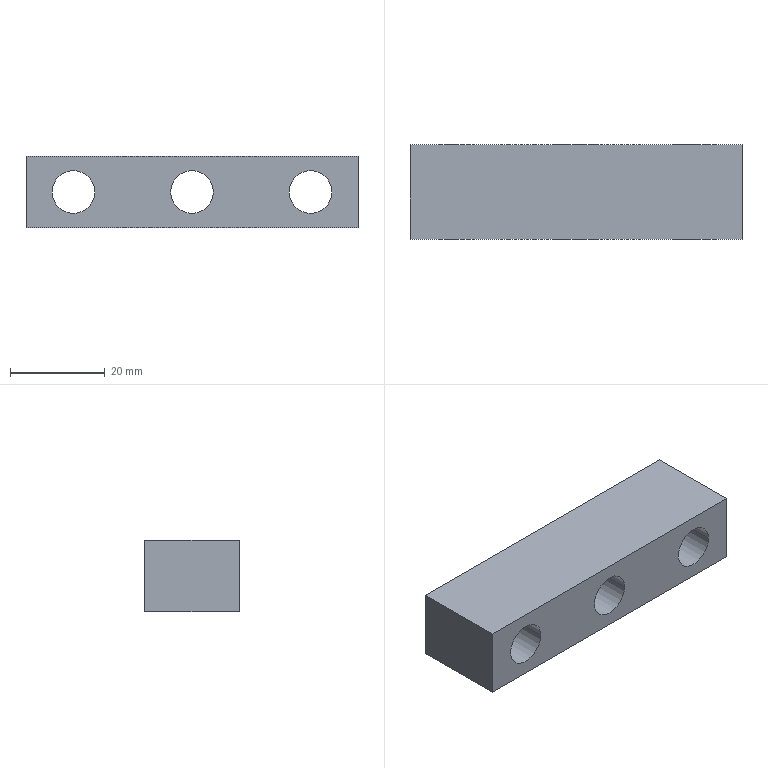Component | SolidWorks | -SpacerPlate-1 | 1 solid | 12 faces | box 70 x 20 x 15 mm | volume 17183 mm3 | cylinder 6 | plane 6 | commonest cylinder face diameters 9 x6
build123d program:
from build123d import *

# Parameters (mm, degrees)
SKETCH1_W                = 15
SKETCH1_H                = 70
BOSS_EXTRUDE1_DEPTH      = 20
F_9_0_9_DIAMETER_HOLE1_D = 9


with BuildPart() as part:
    # Sketch1 → Boss-Extrude1 (new body)
    with BuildSketch(Plane(origin=(0, 0, 0), x_dir=(1, 0, 0), z_dir=(0, 1, 0))):
        with Locations((-7.5, -35)):
            Rectangle(SKETCH1_W, SKETCH1_H)
    extrude(amount=BOSS_EXTRUDE1_DEPTH)

    # 9.0 _9_ Diameter Hole1 (through all)
    with Locations(Plane(origin=(0, 20, 0), x_dir=(1, 0, 0), z_dir=(0, 1, 0))):
        with Locations((-7.5, -10), (-7.5, -35), (-7.5, -60)):
            Hole(F_9_0_9_DIAMETER_HOLE1_D / 2)


solid = part.part

# Placed as in the assembly
solid = solid.moved(Location((170, 1289.5, -85), (0, 90, 0)))
STEP:
#1=COLOUR_RGB('',0.7922,0.8196,0.9333);
#2=FILL_AREA_STYLE_COLOUR('',#1);
#3=FILL_AREA_STYLE('',(#2));
#4=SURFACE_STYLE_FILL_AREA(#3);
#5=SURFACE_SIDE_STYLE('',(#4));
#6=SURFACE_STYLE_USAGE(.BOTH.,#5);
#7=PRESENTATION_STYLE_ASSIGNMENT((#6));
#8=CARTESIAN_POINT('',(9.232,50.768,-3.051));
#9=VERTEX_POINT('',#8);
#10=CARTESIAN_POINT('',(8.878,50.768,-3.051));
#11=VERTEX_POINT('',#10);
#12=CARTESIAN_POINT('',(9.055,50.768,-3.051));
#13=DIRECTION('',(0.,1.,0.));
#14=DIRECTION('',(-1.,0.,0.));
#15=AXIS2_PLACEMENT_3D('',#12,#13,#14);
#16=CIRCLE('',#15,0.1772);
#17=EDGE_CURVE('',#9,#11,#16,.T.);
#18=ORIENTED_EDGE('',*,*,#17,.F.);
#19=CARTESIAN_POINT('',(9.232,51.555,-3.051));
#20=VERTEX_POINT('',#19);
#21=CARTESIAN_POINT('',(9.232,51.555,-3.051));
#22=DIRECTION('',(0.,1.,0.));
#23=VECTOR('',#22,39.37);
#24=LINE('',#21,#23);
#25=EDGE_CURVE('',#9,#20,#24,.T.);
#26=ORIENTED_EDGE('',*,*,#25,.T.);
#27=CARTESIAN_POINT('',(8.878,51.555,-3.051));
#28=VERTEX_POINT('',#27);
#29=CARTESIAN_POINT('',(9.055,51.555,-3.051));
#30=DIRECTION('',(0.,1.,0.));
#31=DIRECTION('',(-1.,0.,0.));
#32=AXIS2_PLACEMENT_3D('',#29,#30,#31);
#33=CIRCLE('',#32,0.1772);
#34=EDGE_CURVE('',#20,#28,#33,.T.);
#35=ORIENTED_EDGE('',*,*,#34,.T.);
#36=CARTESIAN_POINT('',(8.878,51.555,-3.051));
#37=DIRECTION('',(0.,1.,0.));
#38=VECTOR('',#37,39.37);
#39=LINE('',#36,#38);
#40=EDGE_CURVE('',#11,#28,#39,.T.);
#41=ORIENTED_EDGE('',*,*,#40,.F.);
#42=EDGE_LOOP('',(#18,#26,#35,#41));
#43=FACE_OUTER_BOUND('',#42,.T.);
#44=CARTESIAN_POINT('',(9.055,51.555,-3.051));
#45=DIRECTION('',(0.,1.,0.));
#46=DIRECTION('',(-1.,0.,0.));
#47=AXIS2_PLACEMENT_3D('',#44,#45,#46);
#48=CYLINDRICAL_SURFACE('',#47,0.1772);
#49=ADVANCED_FACE('',(#43),#48,.F.);
#50=CARTESIAN_POINT('',(8.248,50.768,-3.051));
#51=VERTEX_POINT('',#50);
#52=CARTESIAN_POINT('',(7.894,50.768,-3.051));
#53=VERTEX_POINT('',#52);
#54=CARTESIAN_POINT('',(8.071,50.768,-3.051));
#55=DIRECTION('',(0.,1.,0.));
#56=DIRECTION('',(-1.,0.,0.));
#57=AXIS2_PLACEMENT_3D('',#54,#55,#56);
#58=CIRCLE('',#57,0.1772);
#59=EDGE_CURVE('',#51,#53,#58,.T.);
#60=ORIENTED_EDGE('',*,*,#59,.F.);
#61=CARTESIAN_POINT('',(8.248,51.555,-3.051));
#62=VERTEX_POINT('',#61);
#63=CARTESIAN_POINT('',(8.248,51.555,-3.051));
#64=DIRECTION('',(0.,1.,0.));
#65=VECTOR('',#64,39.37);
#66=LINE('',#63,#65);
#67=EDGE_CURVE('',#51,#62,#66,.T.);
#68=ORIENTED_EDGE('',*,*,#67,.T.);
#69=CARTESIAN_POINT('',(7.894,51.555,-3.051));
#70=VERTEX_POINT('',#69);
#71=CARTESIAN_POINT('',(8.071,51.555,-3.051));
#72=DIRECTION('',(0.,1.,0.));
#73=DIRECTION('',(-1.,0.,0.));
#74=AXIS2_PLACEMENT_3D('',#71,#72,#73);
#75=CIRCLE('',#74,0.1772);
#76=EDGE_CURVE('',#62,#70,#75,.T.);
#77=ORIENTED_EDGE('',*,*,#76,.T.);
#78=CARTESIAN_POINT('',(7.894,51.555,-3.051));
#79=DIRECTION('',(0.,1.,0.));
#80=VECTOR('',#79,39.37);
#81=LINE('',#78,#80);
#82=EDGE_CURVE('',#53,#70,#81,.T.);
#83=ORIENTED_EDGE('',*,*,#82,.F.);
#84=EDGE_LOOP('',(#60,#68,#77,#83));
#85=FACE_OUTER_BOUND('',#84,.T.);
#86=CARTESIAN_POINT('',(8.071,51.555,-3.051));
#87=DIRECTION('',(0.,1.,0.));
#88=DIRECTION('',(-1.,0.,0.));
#89=AXIS2_PLACEMENT_3D('',#86,#87,#88);
#90=CYLINDRICAL_SURFACE('',#89,0.1772);
#91=ADVANCED_FACE('',(#85),#90,.F.);
#92=CARTESIAN_POINT('',(7.264,50.768,-3.051));
#93=VERTEX_POINT('',#92);
#94=CARTESIAN_POINT('',(6.909,50.768,-3.051));
#95=VERTEX_POINT('',#94);
#96=CARTESIAN_POINT('',(7.087,50.768,-3.051));
#97=DIRECTION('',(0.,1.,0.));
#98=DIRECTION('',(-1.,0.,0.));
#99=AXIS2_PLACEMENT_3D('',#96,#97,#98);
#100=CIRCLE('',#99,0.1772);
#101=EDGE_CURVE('',#93,#95,#100,.T.);
#102=ORIENTED_EDGE('',*,*,#101,.F.);
#103=CARTESIAN_POINT('',(7.264,51.555,-3.051));
#104=VERTEX_POINT('',#103);
#105=CARTESIAN_POINT('',(7.264,51.555,-3.051));
#106=DIRECTION('',(0.,1.,0.));
#107=VECTOR('',#106,39.37);
#108=LINE('',#105,#107);
#109=EDGE_CURVE('',#93,#104,#108,.T.);
#110=ORIENTED_EDGE('',*,*,#109,.T.);
#111=CARTESIAN_POINT('',(6.909,51.555,-3.051));
#112=VERTEX_POINT('',#111);
#113=CARTESIAN_POINT('',(7.087,51.555,-3.051));
#114=DIRECTION('',(0.,1.,0.));
#115=DIRECTION('',(-1.,0.,0.));
#116=AXIS2_PLACEMENT_3D('',#113,#114,#115);
#117=CIRCLE('',#116,0.1772);
#118=EDGE_CURVE('',#104,#112,#117,.T.);
#119=ORIENTED_EDGE('',*,*,#118,.T.);
#120=CARTESIAN_POINT('',(6.909,51.555,-3.051));
#121=DIRECTION('',(0.,1.,0.));
#122=VECTOR('',#121,39.37);
#123=LINE('',#120,#122);
#124=EDGE_CURVE('',#95,#112,#123,.T.);
#125=ORIENTED_EDGE('',*,*,#124,.F.);
#126=EDGE_LOOP('',(#102,#110,#119,#125));
#127=FACE_OUTER_BOUND('',#126,.T.);
#128=CARTESIAN_POINT('',(7.087,51.555,-3.051));
#129=DIRECTION('',(0.,1.,0.));
#130=DIRECTION('',(-1.,0.,0.));
#131=AXIS2_PLACEMENT_3D('',#128,#129,#130);
#132=CYLINDRICAL_SURFACE('',#131,0.1772);
#133=ADVANCED_FACE('',(#127),#132,.F.);
#134=CARTESIAN_POINT('',(6.693,50.768,-2.756));
#135=VERTEX_POINT('',#134);
#136=CARTESIAN_POINT('',(9.449,50.768,-2.756));
#137=VERTEX_POINT('',#136);
#138=CARTESIAN_POINT('',(9.449,50.768,-2.756));
#139=DIRECTION('',(1.,0.,-0.));
#140=VECTOR('',#139,39.37);
#141=LINE('',#138,#140);
#142=EDGE_CURVE('',#135,#137,#141,.T.);
#143=ORIENTED_EDGE('',*,*,#142,.T.);
#144=CARTESIAN_POINT('',(9.449,51.555,-2.756));
#145=VERTEX_POINT('',#144);
#146=CARTESIAN_POINT('',(9.449,51.555,-2.756));
#147=DIRECTION('',(0.,-1.,0.));
#148=VECTOR('',#147,39.37);
#149=LINE('',#146,#148);
#150=EDGE_CURVE('',#145,#137,#149,.T.);
#151=ORIENTED_EDGE('',*,*,#150,.F.);
#152=CARTESIAN_POINT('',(6.693,51.555,-2.756));
#153=VERTEX_POINT('',#152);
#154=CARTESIAN_POINT('',(9.449,51.555,-2.756));
#155=DIRECTION('',(1.,0.,-0.));
#156=VECTOR('',#155,39.37);
#157=LINE('',#154,#156);
#158=EDGE_CURVE('',#153,#145,#157,.T.);
#159=ORIENTED_EDGE('',*,*,#158,.F.);
#160=CARTESIAN_POINT('',(6.693,51.555,-2.756));
#161=DIRECTION('',(0.,-1.,0.));
#162=VECTOR('',#161,39.37);
#163=LINE('',#160,#162);
#164=EDGE_CURVE('',#153,#135,#163,.T.);
#165=ORIENTED_EDGE('',*,*,#164,.T.);
#166=EDGE_LOOP('',(#143,#151,#159,#165));
#167=FACE_OUTER_BOUND('',#166,.T.);
#168=CARTESIAN_POINT('',(9.449,51.555,-2.756));
#169=DIRECTION('',(-0.,0.,-1.));
#170=DIRECTION('',(-1.,0.,0.));
#171=AXIS2_PLACEMENT_3D('',#168,#169,#170);
#172=PLANE('',#171);
#173=ADVANCED_FACE('',(#167),#172,.F.);
#174=CARTESIAN_POINT('',(9.449,50.768,-3.346));
#175=VERTEX_POINT('',#174);
#176=CARTESIAN_POINT('',(9.449,50.768,-2.756));
#177=DIRECTION('',(0.,0.,-1.));
#178=VECTOR('',#177,39.37);
#179=LINE('',#176,#178);
#180=EDGE_CURVE('',#137,#175,#179,.T.);
#181=ORIENTED_EDGE('',*,*,#180,.T.);
#182=CARTESIAN_POINT('',(9.449,51.555,-3.346));
#183=VERTEX_POINT('',#182);
#184=CARTESIAN_POINT('',(9.449,51.555,-3.346));
#185=DIRECTION('',(0.,-1.,0.));
#186=VECTOR('',#185,39.37);
#187=LINE('',#184,#186);
#188=EDGE_CURVE('',#183,#175,#187,.T.);
#189=ORIENTED_EDGE('',*,*,#188,.F.);
#190=CARTESIAN_POINT('',(9.449,51.555,-2.756));
#191=DIRECTION('',(0.,0.,-1.));
#192=VECTOR('',#191,39.37);
#193=LINE('',#190,#192);
#194=EDGE_CURVE('',#145,#183,#193,.T.);
#195=ORIENTED_EDGE('',*,*,#194,.F.);
#196=ORIENTED_EDGE('',*,*,#150,.T.);
#197=EDGE_LOOP('',(#181,#189,#195,#196));
#198=FACE_OUTER_BOUND('',#197,.T.);
#199=CARTESIAN_POINT('',(9.449,51.555,-2.756));
#200=DIRECTION('',(-1.,0.,0.));
#201=DIRECTION('',(0.,0.,1.));
#202=AXIS2_PLACEMENT_3D('',#199,#200,#201);
#203=PLANE('',#202);
#204=ADVANCED_FACE('',(#198),#203,.F.);
#205=CARTESIAN_POINT('',(6.693,50.768,-3.346));
#206=VERTEX_POINT('',#205);
#207=CARTESIAN_POINT('',(9.449,50.768,-3.346));
#208=DIRECTION('',(-1.,0.,0.));
#209=VECTOR('',#208,39.37);
#210=LINE('',#207,#209);
#211=EDGE_CURVE('',#175,#206,#210,.T.);
#212=ORIENTED_EDGE('',*,*,#211,.T.);
#213=CARTESIAN_POINT('',(6.693,51.555,-3.346));
#214=VERTEX_POINT('',#213);
#215=CARTESIAN_POINT('',(6.693,51.555,-3.346));
#216=DIRECTION('',(0.,-1.,0.));
#217=VECTOR('',#216,39.37);
#218=LINE('',#215,#217);
#219=EDGE_CURVE('',#214,#206,#218,.T.);
#220=ORIENTED_EDGE('',*,*,#219,.F.);
#221=CARTESIAN_POINT('',(9.449,51.555,-3.346));
#222=DIRECTION('',(-1.,0.,0.));
#223=VECTOR('',#222,39.37);
#224=LINE('',#221,#223);
#225=EDGE_CURVE('',#183,#214,#224,.T.);
#226=ORIENTED_EDGE('',*,*,#225,.F.);
#227=ORIENTED_EDGE('',*,*,#188,.T.);
#228=EDGE_LOOP('',(#212,#220,#226,#227));
#229=FACE_OUTER_BOUND('',#228,.T.);
#230=CARTESIAN_POINT('',(9.449,51.555,-3.346));
#231=DIRECTION('',(0.,0.,1.));
#232=DIRECTION('',(1.,0.,-0.));
#233=AXIS2_PLACEMENT_3D('',#230,#231,#232);
#234=PLANE('',#233);
#235=ADVANCED_FACE('',(#229),#234,.F.);
#236=CARTESIAN_POINT('',(6.693,50.768,-2.756));
#237=DIRECTION('',(0.,0.,1.));
#238=VECTOR('',#237,39.37);
#239=LINE('',#236,#238);
#240=EDGE_CURVE('',#206,#135,#239,.T.);
#241=ORIENTED_EDGE('',*,*,#240,.T.);
#242=ORIENTED_EDGE('',*,*,#164,.F.);
#243=CARTESIAN_POINT('',(6.693,51.555,-2.756));
#244=DIRECTION('',(0.,0.,1.));
#245=VECTOR('',#244,39.37);
#246=LINE('',#243,#245);
#247=EDGE_CURVE('',#214,#153,#246,.T.);
#248=ORIENTED_EDGE('',*,*,#247,.F.);
#249=ORIENTED_EDGE('',*,*,#219,.T.);
#250=EDGE_LOOP('',(#241,#242,#248,#249));
#251=FACE_OUTER_BOUND('',#250,.T.);
#252=CARTESIAN_POINT('',(6.693,51.555,-2.756));
#253=DIRECTION('',(1.,0.,0.));
#254=DIRECTION('',(0.,0.,-1.));
#255=AXIS2_PLACEMENT_3D('',#252,#253,#254);
#256=PLANE('',#255);
#257=ADVANCED_FACE('',(#251),#256,.F.);
#258=CARTESIAN_POINT('',(9.055,51.555,-3.051));
#259=DIRECTION('',(0.,1.,0.));
#260=DIRECTION('',(-1.,0.,0.));
#261=AXIS2_PLACEMENT_3D('',#258,#259,#260);
#262=CIRCLE('',#261,0.1772);
#263=EDGE_CURVE('',#28,#20,#262,.T.);
#264=ORIENTED_EDGE('',*,*,#263,.F.);
#265=ORIENTED_EDGE('',*,*,#34,.F.);
#266=EDGE_LOOP('',(#264,#265));
#267=FACE_BOUND('',#266,.T.);
#268=CARTESIAN_POINT('',(8.071,51.555,-3.051));
#269=DIRECTION('',(0.,1.,0.));
#270=DIRECTION('',(-1.,0.,0.));
#271=AXIS2_PLACEMENT_3D('',#268,#269,#270);
#272=CIRCLE('',#271,0.1772);
#273=EDGE_CURVE('',#70,#62,#272,.T.);
#274=ORIENTED_EDGE('',*,*,#273,.F.);
#275=ORIENTED_EDGE('',*,*,#76,.F.);
#276=EDGE_LOOP('',(#274,#275));
#277=FACE_BOUND('',#276,.T.);
#278=CARTESIAN_POINT('',(7.087,51.555,-3.051));
#279=DIRECTION('',(0.,1.,0.));
#280=DIRECTION('',(-1.,0.,0.));
#281=AXIS2_PLACEMENT_3D('',#278,#279,#280);
#282=CIRCLE('',#281,0.1772);
#283=EDGE_CURVE('',#112,#104,#282,.T.);
#284=ORIENTED_EDGE('',*,*,#283,.F.);
#285=ORIENTED_EDGE('',*,*,#118,.F.);
#286=EDGE_LOOP('',(#284,#285));
#287=FACE_BOUND('',#286,.T.);
#288=ORIENTED_EDGE('',*,*,#158,.T.);
#289=ORIENTED_EDGE('',*,*,#194,.T.);
#290=ORIENTED_EDGE('',*,*,#225,.T.);
#291=ORIENTED_EDGE('',*,*,#247,.T.);
#292=EDGE_LOOP('',(#288,#289,#290,#291));
#293=FACE_OUTER_BOUND('',#292,.T.);
#294=CARTESIAN_POINT('',(9.449,51.555,-2.756));
#295=DIRECTION('',(0.,-1.,0.));
#296=DIRECTION('',(1.,0.,0.));
#297=AXIS2_PLACEMENT_3D('',#294,#295,#296);
#298=PLANE('',#297);
#299=ADVANCED_FACE('',(#267,#277,#287,#293),#298,.F.);
#300=CARTESIAN_POINT('',(9.055,50.768,-3.051));
#301=DIRECTION('',(0.,1.,0.));
#302=DIRECTION('',(-1.,0.,0.));
#303=AXIS2_PLACEMENT_3D('',#300,#301,#302);
#304=CIRCLE('',#303,0.1772);
#305=EDGE_CURVE('',#11,#9,#304,.T.);
#306=ORIENTED_EDGE('',*,*,#305,.T.);
#307=ORIENTED_EDGE('',*,*,#17,.T.);
#308=EDGE_LOOP('',(#306,#307));
#309=FACE_BOUND('',#308,.T.);
#310=CARTESIAN_POINT('',(8.071,50.768,-3.051));
#311=DIRECTION('',(0.,1.,0.));
#312=DIRECTION('',(-1.,0.,0.));
#313=AXIS2_PLACEMENT_3D('',#310,#311,#312);
#314=CIRCLE('',#313,0.1772);
#315=EDGE_CURVE('',#53,#51,#314,.T.);
#316=ORIENTED_EDGE('',*,*,#315,.T.);
#317=ORIENTED_EDGE('',*,*,#59,.T.);
#318=EDGE_LOOP('',(#316,#317));
#319=FACE_BOUND('',#318,.T.);
#320=CARTESIAN_POINT('',(7.087,50.768,-3.051));
#321=DIRECTION('',(0.,1.,0.));
#322=DIRECTION('',(-1.,0.,0.));
#323=AXIS2_PLACEMENT_3D('',#320,#321,#322);
#324=CIRCLE('',#323,0.1772);
#325=EDGE_CURVE('',#95,#93,#324,.T.);
#326=ORIENTED_EDGE('',*,*,#325,.T.);
#327=ORIENTED_EDGE('',*,*,#101,.T.);
#328=EDGE_LOOP('',(#326,#327));
#329=FACE_BOUND('',#328,.T.);
#330=ORIENTED_EDGE('',*,*,#142,.F.);
#331=ORIENTED_EDGE('',*,*,#240,.F.);
#332=ORIENTED_EDGE('',*,*,#211,.F.);
#333=ORIENTED_EDGE('',*,*,#180,.F.);
#334=EDGE_LOOP('',(#330,#331,#332,#333));
#335=FACE_OUTER_BOUND('',#334,.T.);
#336=CARTESIAN_POINT('',(9.449,50.768,-2.756));
#337=DIRECTION('',(0.,-1.,0.));
#338=DIRECTION('',(1.,0.,0.));
#339=AXIS2_PLACEMENT_3D('',#336,#337,#338);
#340=PLANE('',#339);
#341=ADVANCED_FACE('',(#309,#319,#329,#335),#340,.T.);
#342=ORIENTED_EDGE('',*,*,#109,.F.);
#343=ORIENTED_EDGE('',*,*,#325,.F.);
#344=ORIENTED_EDGE('',*,*,#124,.T.);
#345=ORIENTED_EDGE('',*,*,#283,.T.);
#346=EDGE_LOOP('',(#342,#343,#344,#345));
#347=FACE_OUTER_BOUND('',#346,.T.);
#348=CARTESIAN_POINT('',(7.087,51.555,-3.051));
#349=DIRECTION('',(0.,1.,0.));
#350=DIRECTION('',(-1.,0.,0.));
#351=AXIS2_PLACEMENT_3D('',#348,#349,#350);
#352=CYLINDRICAL_SURFACE('',#351,0.1772);
#353=ADVANCED_FACE('',(#347),#352,.F.);
#354=ORIENTED_EDGE('',*,*,#67,.F.);
#355=ORIENTED_EDGE('',*,*,#315,.F.);
#356=ORIENTED_EDGE('',*,*,#82,.T.);
#357=ORIENTED_EDGE('',*,*,#273,.T.);
#358=EDGE_LOOP('',(#354,#355,#356,#357));
#359=FACE_OUTER_BOUND('',#358,.T.);
#360=CARTESIAN_POINT('',(8.071,51.555,-3.051));
#361=DIRECTION('',(0.,1.,0.));
#362=DIRECTION('',(-1.,0.,0.));
#363=AXIS2_PLACEMENT_3D('',#360,#361,#362);
#364=CYLINDRICAL_SURFACE('',#363,0.1772);
#365=ADVANCED_FACE('',(#359),#364,.F.);
#366=ORIENTED_EDGE('',*,*,#25,.F.);
#367=ORIENTED_EDGE('',*,*,#305,.F.);
#368=ORIENTED_EDGE('',*,*,#40,.T.);
#369=ORIENTED_EDGE('',*,*,#263,.T.);
#370=EDGE_LOOP('',(#366,#367,#368,#369));
#371=FACE_OUTER_BOUND('',#370,.T.);
#372=CARTESIAN_POINT('',(9.055,51.555,-3.051));
#373=DIRECTION('',(0.,1.,0.));
#374=DIRECTION('',(-1.,0.,0.));
#375=AXIS2_PLACEMENT_3D('',#372,#373,#374);
#376=CYLINDRICAL_SURFACE('',#375,0.1772);
#377=ADVANCED_FACE('',(#371),#376,.F.);
#378=CLOSED_SHELL('',(#49,#91,#133,#173,#204,#235,#257,#299,#341,#353,#365,#377));
#379=MANIFOLD_SOLID_BREP('',#378);
#380=STYLED_ITEM('',(#7),#379);
#381=(LENGTH_UNIT()NAMED_UNIT(*)SI_UNIT($,.METRE.));
#382=LENGTH_MEASURE_WITH_UNIT(LENGTH_MEASURE(0.0254),#381);
#383=DIMENSIONAL_EXPONENTS(1.,0.,0.,0.,0.,0.,0.);
#384=(CONVERSION_BASED_UNIT('',#382)LENGTH_UNIT()NAMED_UNIT(#383));
#385=UNCERTAINTY_MEASURE_WITH_UNIT(LENGTH_MEASURE(0.00001),#384,'','');
#386=(NAMED_UNIT(*)PLANE_ANGLE_UNIT()SI_UNIT($,.RADIAN.));
#387=(NAMED_UNIT(*)SI_UNIT($,.STERADIAN.)SOLID_ANGLE_UNIT());
#388=(GEOMETRIC_REPRESENTATION_CONTEXT(3)GLOBAL_UNCERTAINTY_ASSIGNED_CONTEXT((#385))GLOBAL_UNIT_ASSIGNED_CONTEXT((#384,#386,#387))REPRESENTATION_CONTEXT('',''));
#389=MECHANICAL_DESIGN_GEOMETRIC_PRESENTATION_REPRESENTATION('',(#380),#388);
#390=CARTESIAN_POINT('',(0.,0.,0.));
#391=DIRECTION('',(0.,0.,1.));
#392=DIRECTION('',(1.,0.,0.));
#393=AXIS2_PLACEMENT_3D('',#390,#391,#392);
#394=(LENGTH_UNIT()NAMED_UNIT(*)SI_UNIT($,.METRE.));
#395=LENGTH_MEASURE_WITH_UNIT(LENGTH_MEASURE(0.0254),#394);
#396=DIMENSIONAL_EXPONENTS(1.,0.,0.,0.,0.,0.,0.);
#397=(CONVERSION_BASED_UNIT('',#395)LENGTH_UNIT()NAMED_UNIT(#396));
#398=UNCERTAINTY_MEASURE_WITH_UNIT(LENGTH_MEASURE(0.00001),#397,'','');
#399=(NAMED_UNIT(*)PLANE_ANGLE_UNIT()SI_UNIT($,.RADIAN.));
#400=(NAMED_UNIT(*)SI_UNIT($,.STERADIAN.)SOLID_ANGLE_UNIT());
#401=(GEOMETRIC_REPRESENTATION_CONTEXT(3)GLOBAL_UNCERTAINTY_ASSIGNED_CONTEXT((#398))GLOBAL_UNIT_ASSIGNED_CONTEXT((#397,#399,#400))REPRESENTATION_CONTEXT('',''));
#402=ADVANCED_BREP_SHAPE_REPRESENTATION('',(#379,#393),#401);
#403=PRESENTATION_LAYER_ASSIGNMENT('','',(#380));